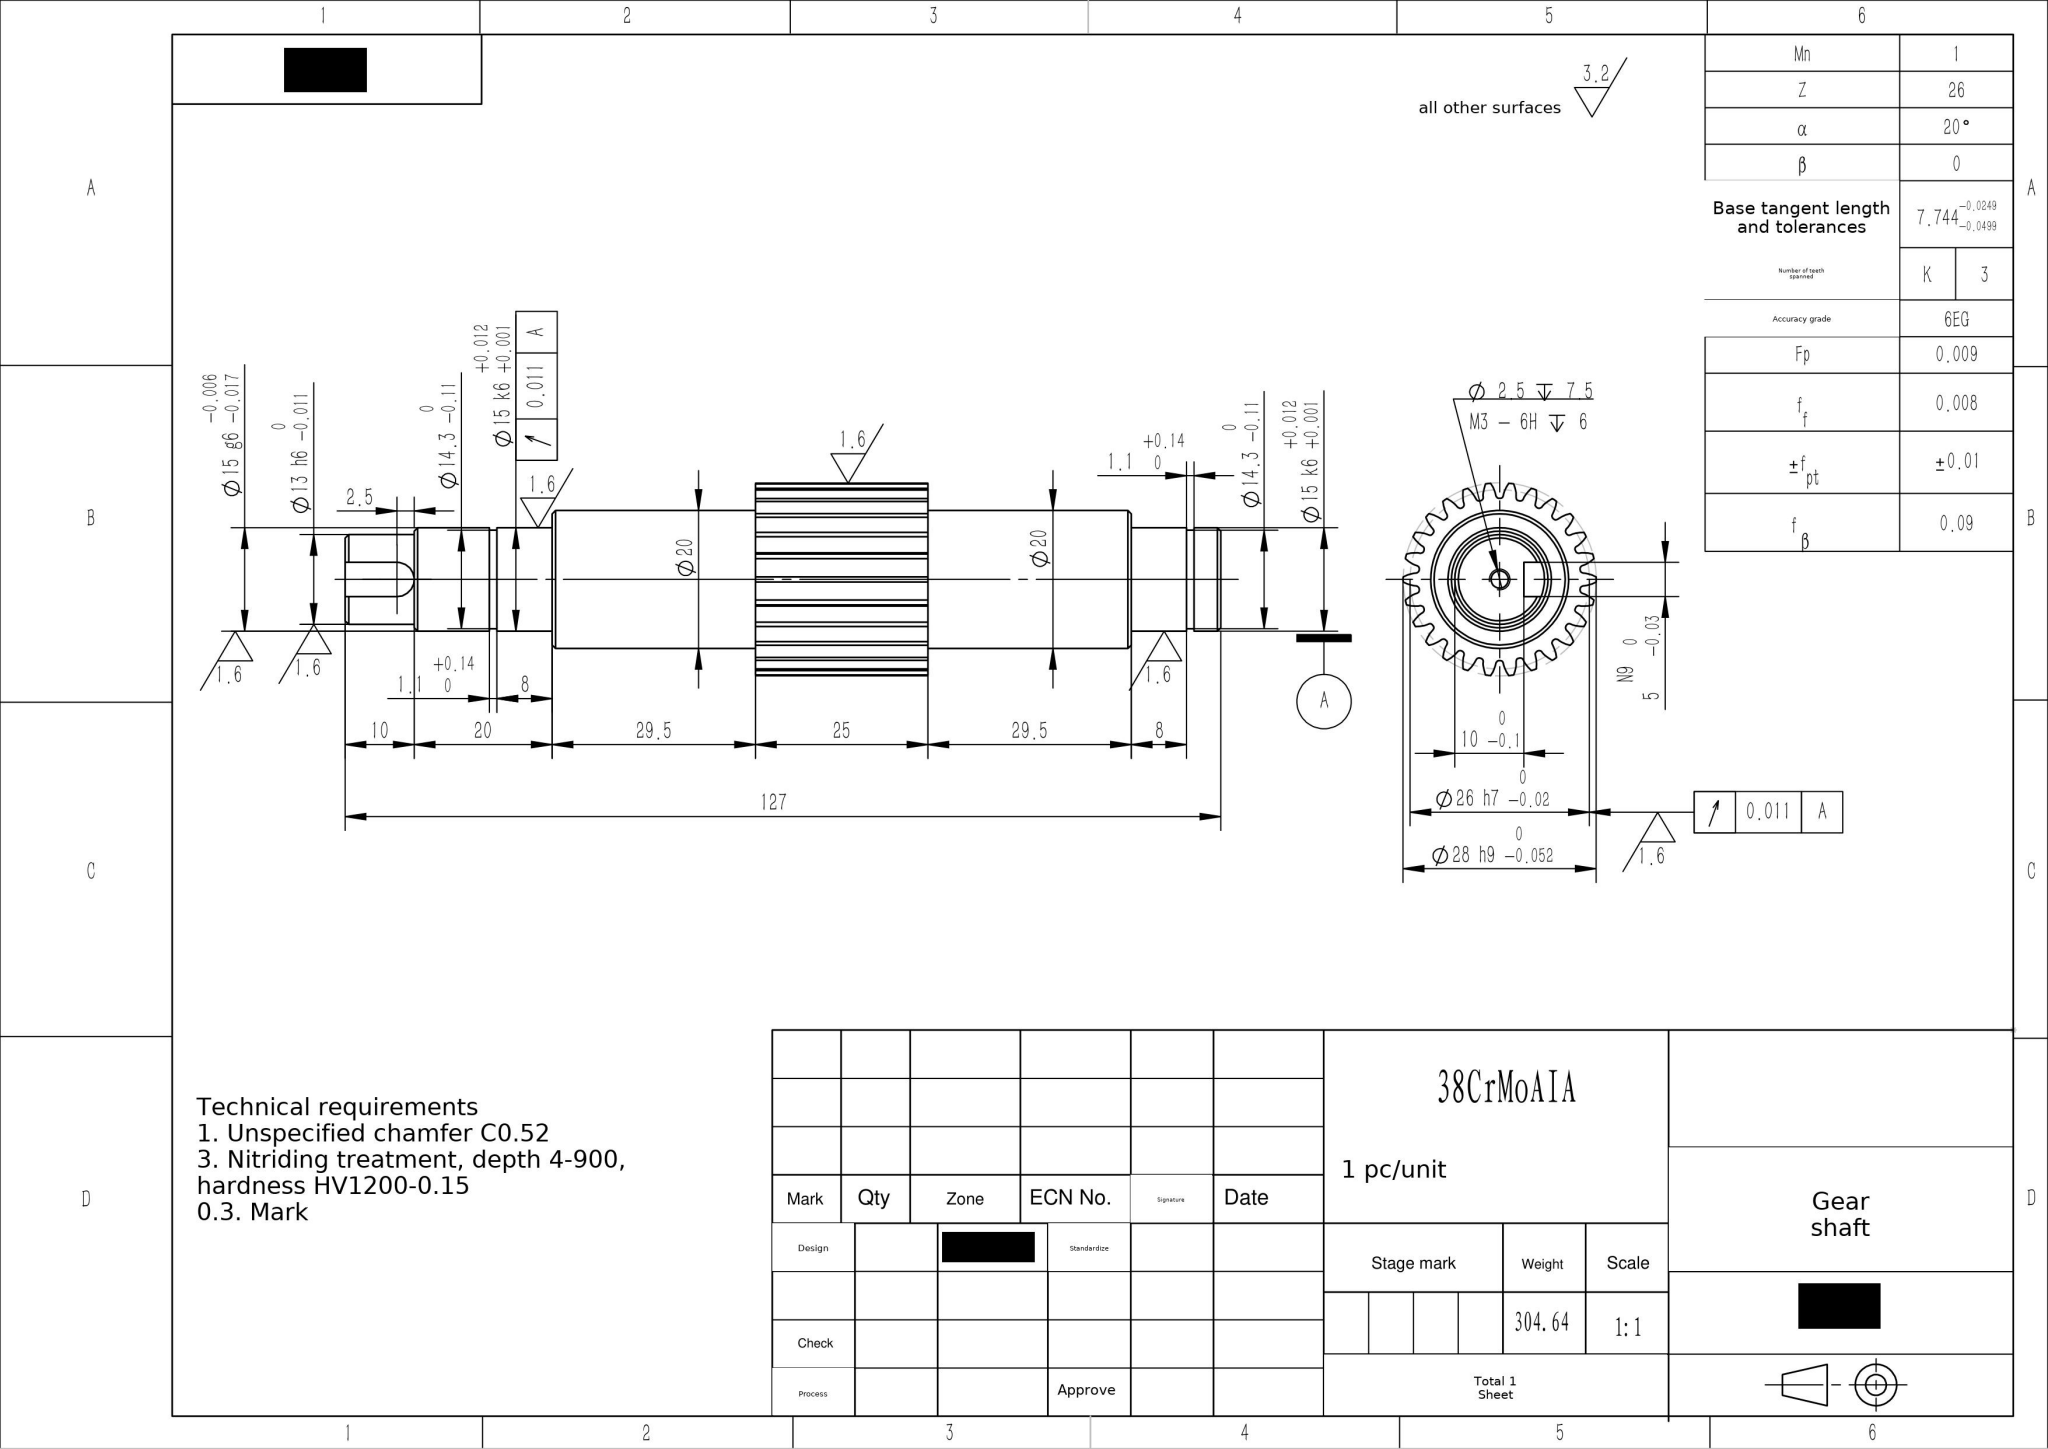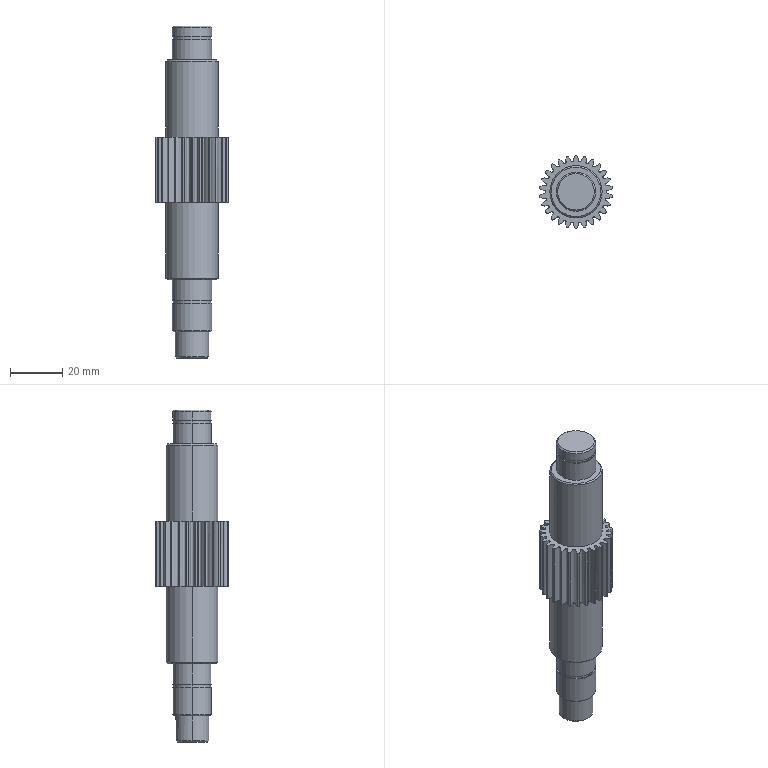Part | SolidWorks | mm | material 38CrMoAlA | 1 solid | 101 faces | box 27.87 x 28 x 127 mm | volume 38558 mm3 | cylinder 48 | spline 26 | plane 14 | cone 13 | commonest cylinder face diameters 28 x26 15 x8 14.3 x4 20 x4 13 x3 2.5 x2 5 x1